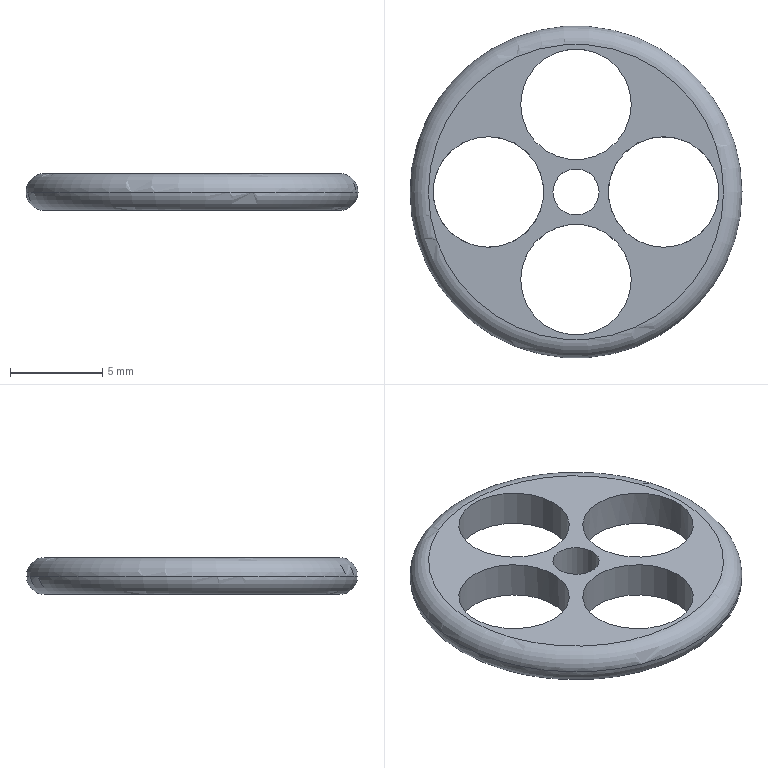Component | NX | ROTARY_SWITCH | 1 solid | 9 faces | volume 249 mm3 | cylinder 5 | plane 2 | torus 2 | commonest cylinder face diameters 6 x4 2.5 x1